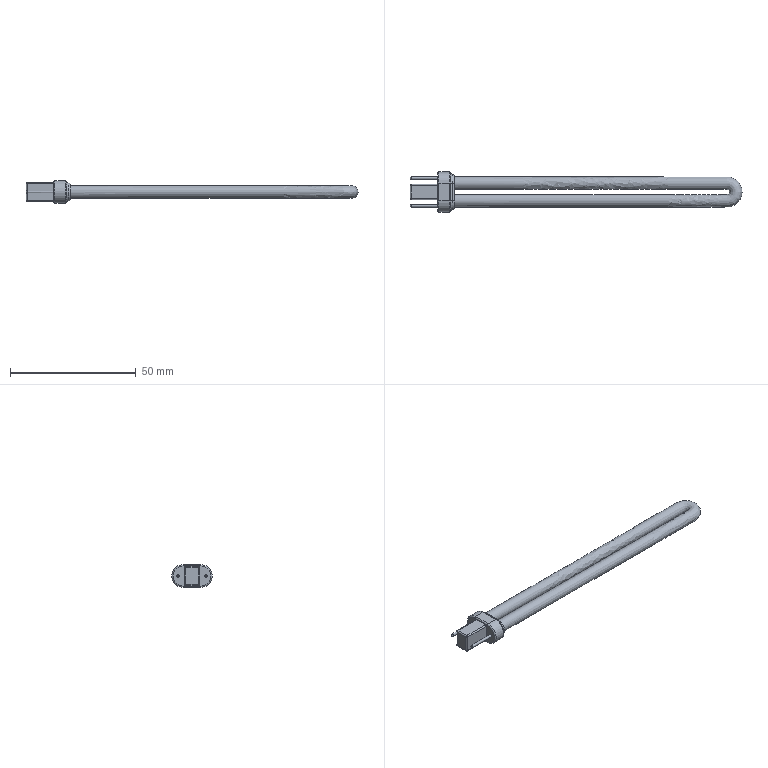Component | NX | DENG | 1 solid | 46 faces | volume 5457 mm3 | cylinder 20 | plane 11 | torus 8 | sphere 4 | spline 3 | commonest cylinder face diameters 1 x16 9 x2 2 x2